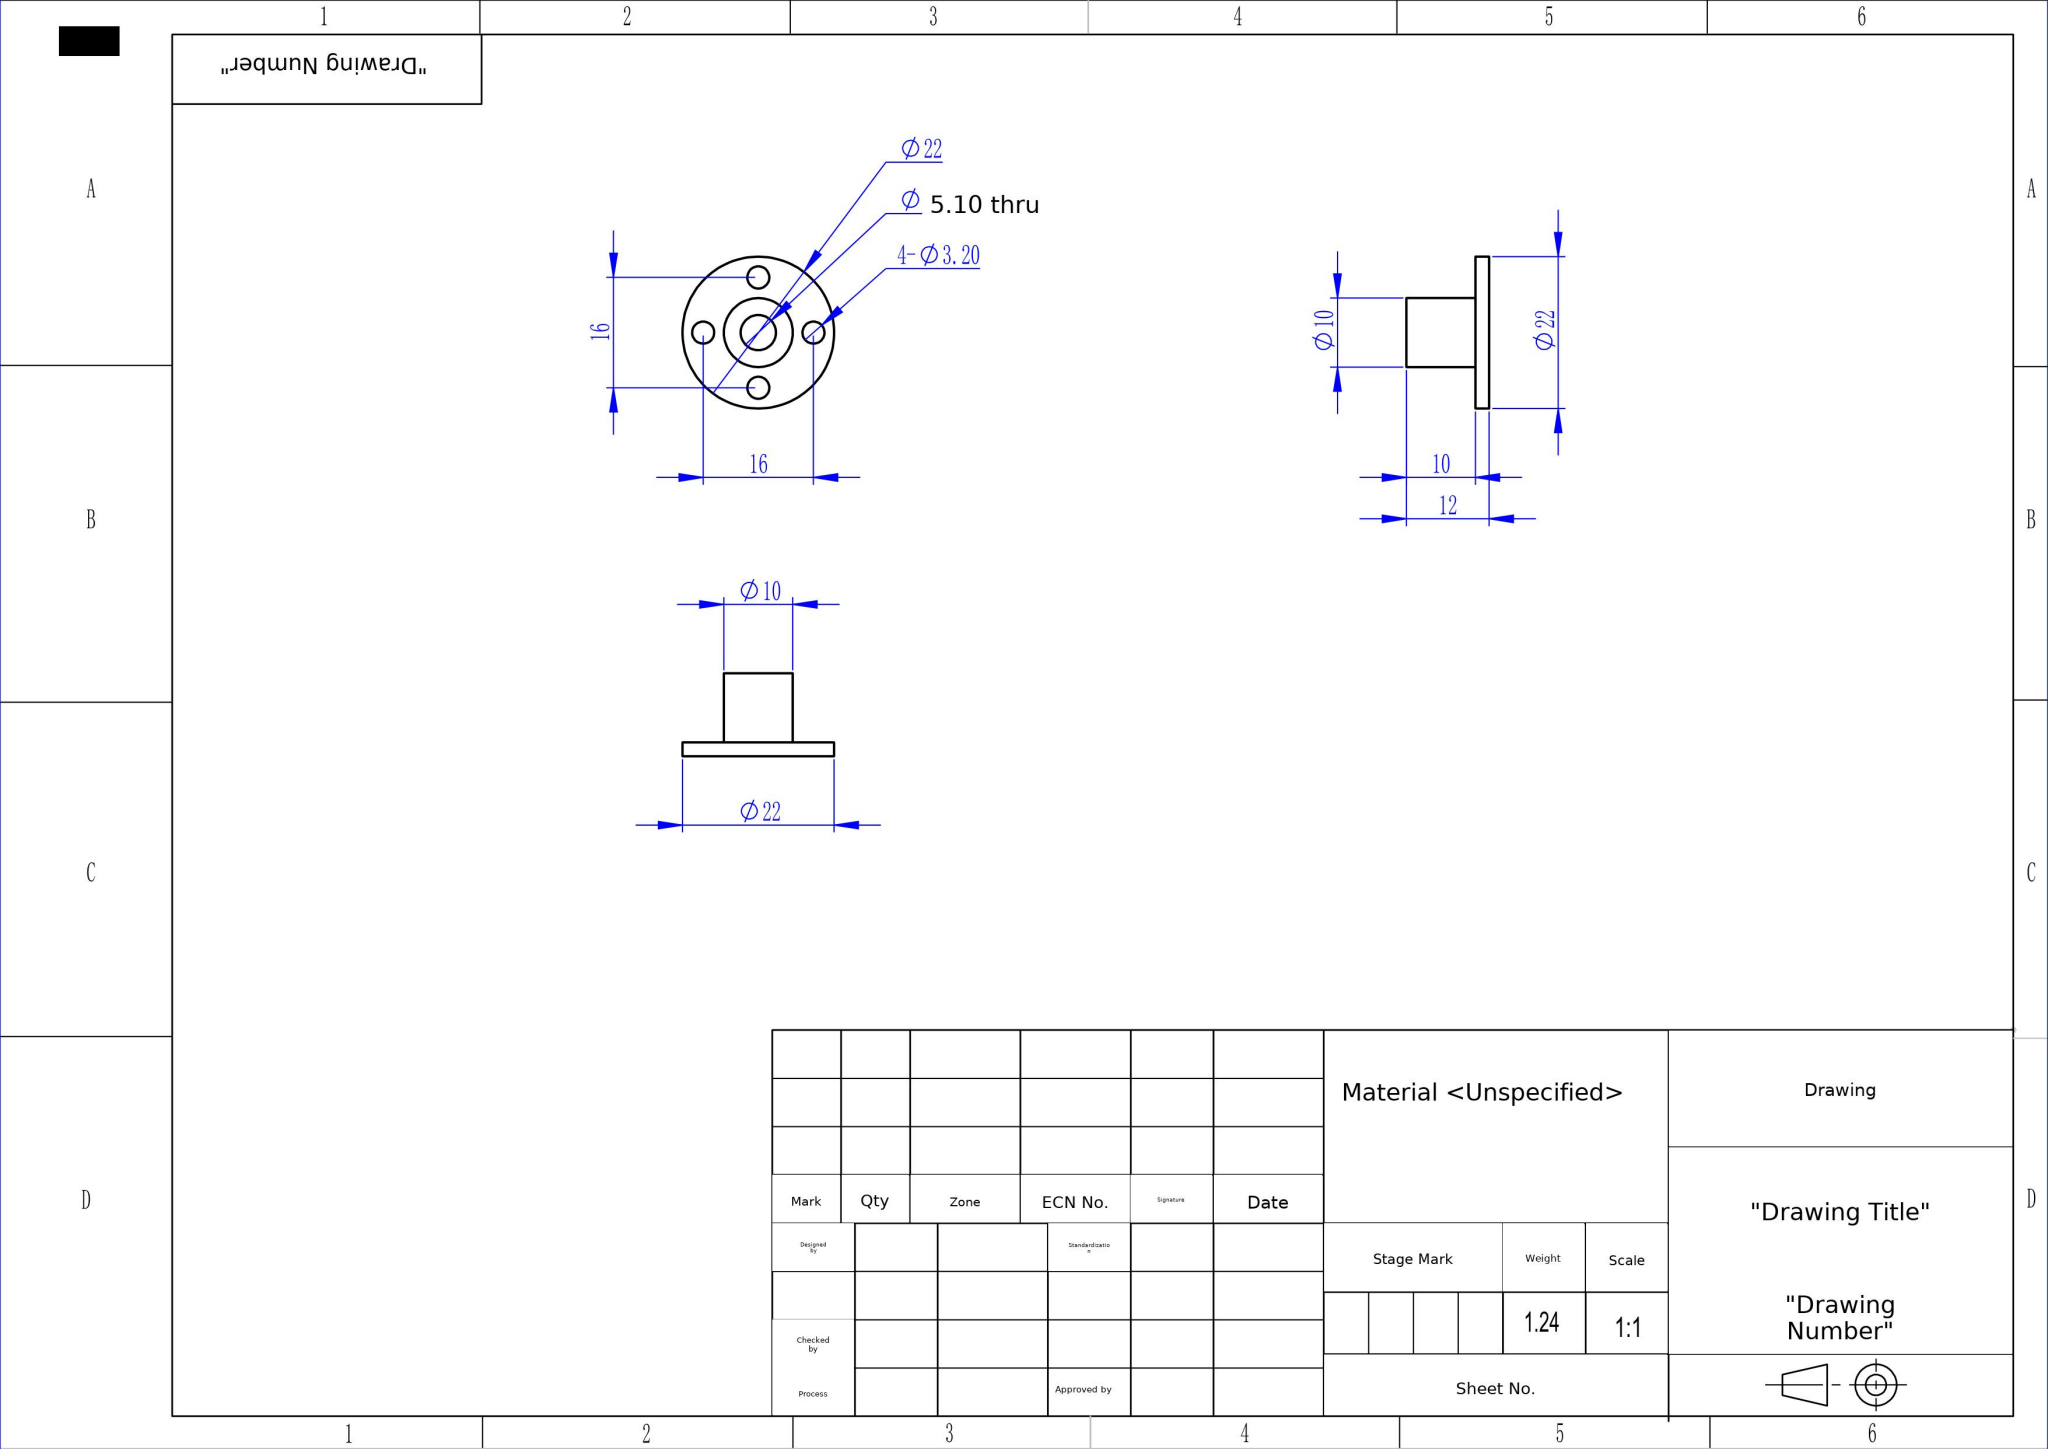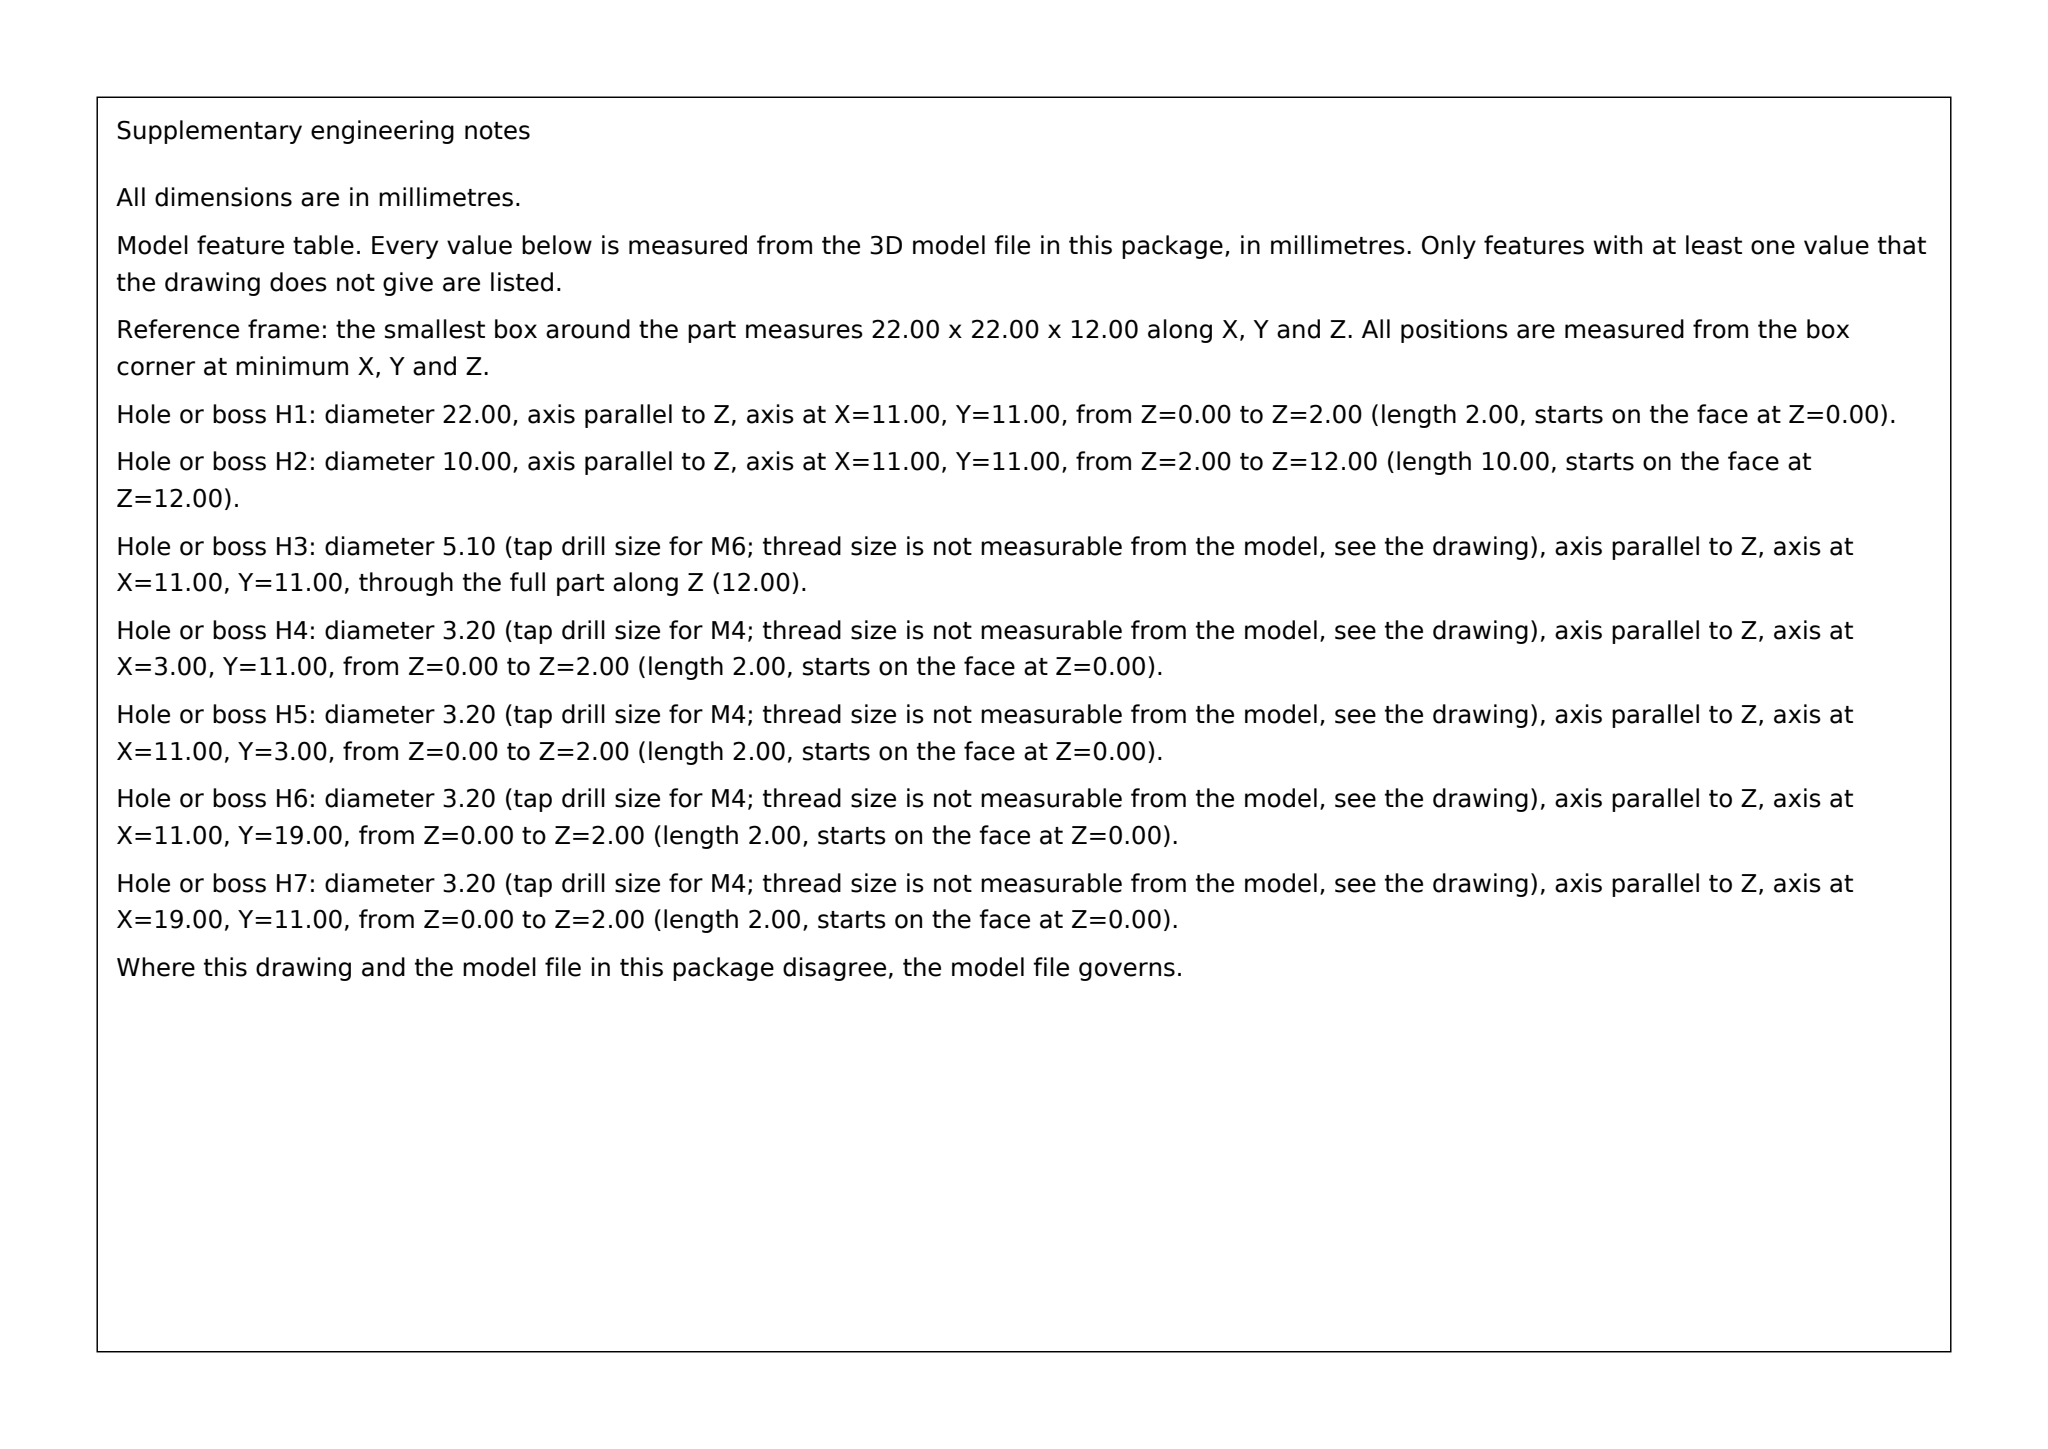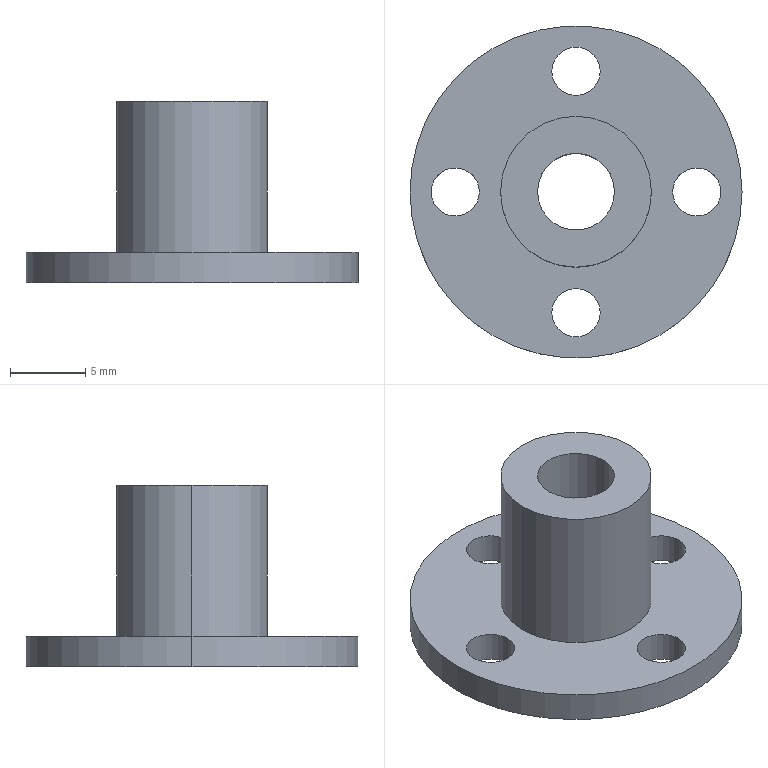Part | SolidWorks | mm | 1 solid | 17 faces | box 22 x 22 x 12 mm | volume 1236 mm3 | cylinder 14 | plane 3 | commonest cylinder face diameters 3.2 x8 5.1 x2 10 x2 22 x2
build123d program:
from build123d import *

# Parameters (mm, degrees)
SKETCH1_R           = 11
SKETCH1_R_2         = 1.6
BOSS_EXTRUDE1_DEPTH = 2
SKETCH2_R           = 5
BOSS_EXTRUDE2_DEPTH = 10
SKETCH3_R           = 2.55
CUT_EXTRUDE1_DEPTH  = 20.647


with BuildPart() as part:
    # Sketch1 → Boss-Extrude1 (new body)
    with BuildSketch(Plane.XY):
        Circle(SKETCH1_R)
        with Locations((-8, 0)):
            Circle(SKETCH1_R_2, mode=Mode.SUBTRACT)
        with Locations((8, 0)):
            Circle(SKETCH1_R_2, mode=Mode.SUBTRACT)
        with Locations((0, -8)):
            Circle(SKETCH1_R_2, mode=Mode.SUBTRACT)
        with Locations((0, 8)):
            Circle(SKETCH1_R_2, mode=Mode.SUBTRACT)
    extrude(amount=BOSS_EXTRUDE1_DEPTH)

    # Sketch2 → Boss-Extrude2 (add)
    with BuildSketch(Plane.XY.offset(2)):
        Circle(SKETCH2_R)
    extrude(amount=BOSS_EXTRUDE2_DEPTH)

    # Sketch3 → Cut-Extrude1 (cut, through all)
    with BuildSketch(Plane.XY.offset(12)):
        Circle(SKETCH3_R)
    extrude(amount=-CUT_EXTRUDE1_DEPTH, mode=Mode.SUBTRACT)


solid = part.part
STEP:
#1=CARTESIAN_POINT('',(-2.55,0.,0.));
#2=VERTEX_POINT('',#1);
#3=CARTESIAN_POINT('',(2.55,0.,0.));
#4=VERTEX_POINT('',#3);
#5=CARTESIAN_POINT('',(0.,0.,0.));
#6=DIRECTION('',(0.,0.,1.));
#7=DIRECTION('',(1.,0.,0.));
#8=AXIS2_PLACEMENT_3D('',#5,#6,#7);
#9=CIRCLE('',#8,2.55);
#10=EDGE_CURVE('',#2,#4,#9,.T.);
#11=ORIENTED_EDGE('',*,*,#10,.F.);
#12=CARTESIAN_POINT('',(-2.55,0.,12.));
#13=VERTEX_POINT('',#12);
#14=CARTESIAN_POINT('',(-2.55,0.,0.));
#15=DIRECTION('',(0.,0.,1.));
#16=VECTOR('',#15,1000.);
#17=LINE('',#14,#16);
#18=EDGE_CURVE('',#2,#13,#17,.T.);
#19=ORIENTED_EDGE('',*,*,#18,.T.);
#20=CARTESIAN_POINT('',(2.55,0.,12.));
#21=VERTEX_POINT('',#20);
#22=CARTESIAN_POINT('',(0.,0.,12.));
#23=DIRECTION('',(0.,0.,1.));
#24=DIRECTION('',(1.,0.,0.));
#25=AXIS2_PLACEMENT_3D('',#22,#23,#24);
#26=CIRCLE('',#25,2.55);
#27=EDGE_CURVE('',#13,#21,#26,.T.);
#28=ORIENTED_EDGE('',*,*,#27,.T.);
#29=CARTESIAN_POINT('',(2.55,0.,0.));
#30=DIRECTION('',(0.,0.,1.));
#31=VECTOR('',#30,1000.);
#32=LINE('',#29,#31);
#33=EDGE_CURVE('',#4,#21,#32,.T.);
#34=ORIENTED_EDGE('',*,*,#33,.F.);
#35=EDGE_LOOP('',(#11,#19,#28,#34));
#36=FACE_OUTER_BOUND('',#35,.T.);
#37=CARTESIAN_POINT('',(0.,0.,0.));
#38=DIRECTION('',(0.,0.,1.));
#39=DIRECTION('',(1.,0.,0.));
#40=AXIS2_PLACEMENT_3D('',#37,#38,#39);
#41=CYLINDRICAL_SURFACE('',#40,2.55);
#42=ADVANCED_FACE('',(#36),#41,.F.);
#43=CARTESIAN_POINT('',(5.,0.,12.));
#44=VERTEX_POINT('',#43);
#45=CARTESIAN_POINT('',(-5.,0.,12.));
#46=VERTEX_POINT('',#45);
#47=CARTESIAN_POINT('',(0.,0.,12.));
#48=DIRECTION('',(0.,0.,1.));
#49=DIRECTION('',(1.,0.,0.));
#50=AXIS2_PLACEMENT_3D('',#47,#48,#49);
#51=CIRCLE('',#50,5.);
#52=EDGE_CURVE('',#44,#46,#51,.T.);
#53=ORIENTED_EDGE('',*,*,#52,.F.);
#54=CARTESIAN_POINT('',(5.,0.,2.));
#55=VERTEX_POINT('',#54);
#56=CARTESIAN_POINT('',(5.,0.,12.));
#57=DIRECTION('',(0.,0.,-1.));
#58=VECTOR('',#57,1000.);
#59=LINE('',#56,#58);
#60=EDGE_CURVE('',#44,#55,#59,.T.);
#61=ORIENTED_EDGE('',*,*,#60,.T.);
#62=CARTESIAN_POINT('',(-5.,0.,2.));
#63=VERTEX_POINT('',#62);
#64=CARTESIAN_POINT('',(0.,0.,2.));
#65=DIRECTION('',(0.,0.,1.));
#66=DIRECTION('',(1.,0.,0.));
#67=AXIS2_PLACEMENT_3D('',#64,#65,#66);
#68=CIRCLE('',#67,5.);
#69=EDGE_CURVE('',#55,#63,#68,.T.);
#70=ORIENTED_EDGE('',*,*,#69,.T.);
#71=CARTESIAN_POINT('',(-5.,0.,12.));
#72=DIRECTION('',(0.,0.,-1.));
#73=VECTOR('',#72,1000.);
#74=LINE('',#71,#73);
#75=EDGE_CURVE('',#46,#63,#74,.T.);
#76=ORIENTED_EDGE('',*,*,#75,.F.);
#77=EDGE_LOOP('',(#53,#61,#70,#76));
#78=FACE_OUTER_BOUND('',#77,.T.);
#79=CARTESIAN_POINT('',(0.,0.,12.));
#80=DIRECTION('',(0.,0.,-1.));
#81=DIRECTION('',(-1.,0.,0.));
#82=AXIS2_PLACEMENT_3D('',#79,#80,#81);
#83=CYLINDRICAL_SURFACE('',#82,5.);
#84=ADVANCED_FACE('',(#78),#83,.T.);
#85=CARTESIAN_POINT('',(-1.6,8.,2.));
#86=VERTEX_POINT('',#85);
#87=CARTESIAN_POINT('',(1.6,8.,2.));
#88=VERTEX_POINT('',#87);
#89=CARTESIAN_POINT('',(0.,8.,2.));
#90=DIRECTION('',(0.,0.,1.));
#91=DIRECTION('',(1.,0.,0.));
#92=AXIS2_PLACEMENT_3D('',#89,#90,#91);
#93=CIRCLE('',#92,1.6);
#94=EDGE_CURVE('',#86,#88,#93,.T.);
#95=ORIENTED_EDGE('',*,*,#94,.T.);
#96=CARTESIAN_POINT('',(1.6,8.,0.));
#97=VERTEX_POINT('',#96);
#98=CARTESIAN_POINT('',(1.6,8.,2.));
#99=DIRECTION('',(0.,0.,-1.));
#100=VECTOR('',#99,1000.);
#101=LINE('',#98,#100);
#102=EDGE_CURVE('',#88,#97,#101,.T.);
#103=ORIENTED_EDGE('',*,*,#102,.T.);
#104=CARTESIAN_POINT('',(-1.6,8.,0.));
#105=VERTEX_POINT('',#104);
#106=CARTESIAN_POINT('',(0.,8.,0.));
#107=DIRECTION('',(0.,0.,1.));
#108=DIRECTION('',(1.,0.,0.));
#109=AXIS2_PLACEMENT_3D('',#106,#107,#108);
#110=CIRCLE('',#109,1.6);
#111=EDGE_CURVE('',#105,#97,#110,.T.);
#112=ORIENTED_EDGE('',*,*,#111,.F.);
#113=CARTESIAN_POINT('',(-1.6,8.,2.));
#114=DIRECTION('',(0.,0.,-1.));
#115=VECTOR('',#114,1000.);
#116=LINE('',#113,#115);
#117=EDGE_CURVE('',#86,#105,#116,.T.);
#118=ORIENTED_EDGE('',*,*,#117,.F.);
#119=EDGE_LOOP('',(#95,#103,#112,#118));
#120=FACE_OUTER_BOUND('',#119,.T.);
#121=CARTESIAN_POINT('',(0.,8.,2.));
#122=DIRECTION('',(0.,0.,-1.));
#123=DIRECTION('',(-1.,0.,0.));
#124=AXIS2_PLACEMENT_3D('',#121,#122,#123);
#125=CYLINDRICAL_SURFACE('',#124,1.6);
#126=ADVANCED_FACE('',(#120),#125,.F.);
#127=CARTESIAN_POINT('',(-1.6,-8.,2.));
#128=VERTEX_POINT('',#127);
#129=CARTESIAN_POINT('',(1.6,-8.,2.));
#130=VERTEX_POINT('',#129);
#131=CARTESIAN_POINT('',(0.,-8.,2.));
#132=DIRECTION('',(0.,0.,1.));
#133=DIRECTION('',(1.,0.,0.));
#134=AXIS2_PLACEMENT_3D('',#131,#132,#133);
#135=CIRCLE('',#134,1.6);
#136=EDGE_CURVE('',#128,#130,#135,.T.);
#137=ORIENTED_EDGE('',*,*,#136,.T.);
#138=CARTESIAN_POINT('',(1.6,-8.,0.));
#139=VERTEX_POINT('',#138);
#140=CARTESIAN_POINT('',(1.6,-8.,2.));
#141=DIRECTION('',(0.,0.,-1.));
#142=VECTOR('',#141,1000.);
#143=LINE('',#140,#142);
#144=EDGE_CURVE('',#130,#139,#143,.T.);
#145=ORIENTED_EDGE('',*,*,#144,.T.);
#146=CARTESIAN_POINT('',(-1.6,-8.,0.));
#147=VERTEX_POINT('',#146);
#148=CARTESIAN_POINT('',(0.,-8.,0.));
#149=DIRECTION('',(0.,0.,1.));
#150=DIRECTION('',(1.,0.,0.));
#151=AXIS2_PLACEMENT_3D('',#148,#149,#150);
#152=CIRCLE('',#151,1.6);
#153=EDGE_CURVE('',#147,#139,#152,.T.);
#154=ORIENTED_EDGE('',*,*,#153,.F.);
#155=CARTESIAN_POINT('',(-1.6,-8.,2.));
#156=DIRECTION('',(0.,0.,-1.));
#157=VECTOR('',#156,1000.);
#158=LINE('',#155,#157);
#159=EDGE_CURVE('',#128,#147,#158,.T.);
#160=ORIENTED_EDGE('',*,*,#159,.F.);
#161=EDGE_LOOP('',(#137,#145,#154,#160));
#162=FACE_OUTER_BOUND('',#161,.T.);
#163=CARTESIAN_POINT('',(0.,-8.,2.));
#164=DIRECTION('',(0.,0.,-1.));
#165=DIRECTION('',(-1.,0.,0.));
#166=AXIS2_PLACEMENT_3D('',#163,#164,#165);
#167=CYLINDRICAL_SURFACE('',#166,1.6);
#168=ADVANCED_FACE('',(#162),#167,.F.);
#169=CARTESIAN_POINT('',(6.4,0.,2.));
#170=VERTEX_POINT('',#169);
#171=CARTESIAN_POINT('',(9.6,0.,2.));
#172=VERTEX_POINT('',#171);
#173=CARTESIAN_POINT('',(8.,0.,2.));
#174=DIRECTION('',(0.,0.,1.));
#175=DIRECTION('',(1.,0.,0.));
#176=AXIS2_PLACEMENT_3D('',#173,#174,#175);
#177=CIRCLE('',#176,1.6);
#178=EDGE_CURVE('',#170,#172,#177,.T.);
#179=ORIENTED_EDGE('',*,*,#178,.T.);
#180=CARTESIAN_POINT('',(9.6,0.,0.));
#181=VERTEX_POINT('',#180);
#182=CARTESIAN_POINT('',(9.6,0.,2.));
#183=DIRECTION('',(0.,0.,-1.));
#184=VECTOR('',#183,1000.);
#185=LINE('',#182,#184);
#186=EDGE_CURVE('',#172,#181,#185,.T.);
#187=ORIENTED_EDGE('',*,*,#186,.T.);
#188=CARTESIAN_POINT('',(6.4,0.,0.));
#189=VERTEX_POINT('',#188);
#190=CARTESIAN_POINT('',(8.,0.,0.));
#191=DIRECTION('',(0.,0.,1.));
#192=DIRECTION('',(1.,0.,0.));
#193=AXIS2_PLACEMENT_3D('',#190,#191,#192);
#194=CIRCLE('',#193,1.6);
#195=EDGE_CURVE('',#189,#181,#194,.T.);
#196=ORIENTED_EDGE('',*,*,#195,.F.);
#197=CARTESIAN_POINT('',(6.4,0.,2.));
#198=DIRECTION('',(0.,0.,-1.));
#199=VECTOR('',#198,1000.);
#200=LINE('',#197,#199);
#201=EDGE_CURVE('',#170,#189,#200,.T.);
#202=ORIENTED_EDGE('',*,*,#201,.F.);
#203=EDGE_LOOP('',(#179,#187,#196,#202));
#204=FACE_OUTER_BOUND('',#203,.T.);
#205=CARTESIAN_POINT('',(8.,0.,2.));
#206=DIRECTION('',(0.,0.,-1.));
#207=DIRECTION('',(-1.,0.,0.));
#208=AXIS2_PLACEMENT_3D('',#205,#206,#207);
#209=CYLINDRICAL_SURFACE('',#208,1.6);
#210=ADVANCED_FACE('',(#204),#209,.F.);
#211=CARTESIAN_POINT('',(-9.6,0.,2.));
#212=VERTEX_POINT('',#211);
#213=CARTESIAN_POINT('',(-6.4,0.,2.));
#214=VERTEX_POINT('',#213);
#215=CARTESIAN_POINT('',(-8.,0.,2.));
#216=DIRECTION('',(0.,0.,1.));
#217=DIRECTION('',(1.,0.,0.));
#218=AXIS2_PLACEMENT_3D('',#215,#216,#217);
#219=CIRCLE('',#218,1.6);
#220=EDGE_CURVE('',#212,#214,#219,.T.);
#221=ORIENTED_EDGE('',*,*,#220,.T.);
#222=CARTESIAN_POINT('',(-6.4,0.,0.));
#223=VERTEX_POINT('',#222);
#224=CARTESIAN_POINT('',(-6.4,0.,2.));
#225=DIRECTION('',(0.,0.,-1.));
#226=VECTOR('',#225,1000.);
#227=LINE('',#224,#226);
#228=EDGE_CURVE('',#214,#223,#227,.T.);
#229=ORIENTED_EDGE('',*,*,#228,.T.);
#230=CARTESIAN_POINT('',(-9.6,0.,0.));
#231=VERTEX_POINT('',#230);
#232=CARTESIAN_POINT('',(-8.,0.,0.));
#233=DIRECTION('',(0.,0.,1.));
#234=DIRECTION('',(1.,0.,0.));
#235=AXIS2_PLACEMENT_3D('',#232,#233,#234);
#236=CIRCLE('',#235,1.6);
#237=EDGE_CURVE('',#231,#223,#236,.T.);
#238=ORIENTED_EDGE('',*,*,#237,.F.);
#239=CARTESIAN_POINT('',(-9.6,0.,2.));
#240=DIRECTION('',(0.,0.,-1.));
#241=VECTOR('',#240,1000.);
#242=LINE('',#239,#241);
#243=EDGE_CURVE('',#212,#231,#242,.T.);
#244=ORIENTED_EDGE('',*,*,#243,.F.);
#245=EDGE_LOOP('',(#221,#229,#238,#244));
#246=FACE_OUTER_BOUND('',#245,.T.);
#247=CARTESIAN_POINT('',(-8.,0.,2.));
#248=DIRECTION('',(0.,0.,-1.));
#249=DIRECTION('',(-1.,0.,0.));
#250=AXIS2_PLACEMENT_3D('',#247,#248,#249);
#251=CYLINDRICAL_SURFACE('',#250,1.6);
#252=ADVANCED_FACE('',(#246),#251,.F.);
#253=CARTESIAN_POINT('',(11.,0.,2.));
#254=VERTEX_POINT('',#253);
#255=CARTESIAN_POINT('',(-11.,0.,2.));
#256=VERTEX_POINT('',#255);
#257=CARTESIAN_POINT('',(0.,0.,2.));
#258=DIRECTION('',(0.,0.,1.));
#259=DIRECTION('',(1.,0.,0.));
#260=AXIS2_PLACEMENT_3D('',#257,#258,#259);
#261=CIRCLE('',#260,11.);
#262=EDGE_CURVE('',#254,#256,#261,.T.);
#263=ORIENTED_EDGE('',*,*,#262,.F.);
#264=CARTESIAN_POINT('',(11.,0.,0.));
#265=VERTEX_POINT('',#264);
#266=CARTESIAN_POINT('',(11.,0.,2.));
#267=DIRECTION('',(0.,0.,-1.));
#268=VECTOR('',#267,1000.);
#269=LINE('',#266,#268);
#270=EDGE_CURVE('',#254,#265,#269,.T.);
#271=ORIENTED_EDGE('',*,*,#270,.T.);
#272=CARTESIAN_POINT('',(-11.,0.,0.));
#273=VERTEX_POINT('',#272);
#274=CARTESIAN_POINT('',(0.,0.,0.));
#275=DIRECTION('',(0.,0.,1.));
#276=DIRECTION('',(1.,0.,0.));
#277=AXIS2_PLACEMENT_3D('',#274,#275,#276);
#278=CIRCLE('',#277,11.);
#279=EDGE_CURVE('',#265,#273,#278,.T.);
#280=ORIENTED_EDGE('',*,*,#279,.T.);
#281=CARTESIAN_POINT('',(-11.,0.,2.));
#282=DIRECTION('',(0.,0.,-1.));
#283=VECTOR('',#282,1000.);
#284=LINE('',#281,#283);
#285=EDGE_CURVE('',#256,#273,#284,.T.);
#286=ORIENTED_EDGE('',*,*,#285,.F.);
#287=EDGE_LOOP('',(#263,#271,#280,#286));
#288=FACE_OUTER_BOUND('',#287,.T.);
#289=CARTESIAN_POINT('',(0.,0.,2.));
#290=DIRECTION('',(0.,0.,-1.));
#291=DIRECTION('',(-1.,0.,0.));
#292=AXIS2_PLACEMENT_3D('',#289,#290,#291);
#293=CYLINDRICAL_SURFACE('',#292,11.);
#294=ADVANCED_FACE('',(#288),#293,.T.);
#295=CARTESIAN_POINT('',(0.,0.,2.));
#296=DIRECTION('',(0.,0.,1.));
#297=DIRECTION('',(1.,0.,0.));
#298=AXIS2_PLACEMENT_3D('',#295,#296,#297);
#299=CIRCLE('',#298,5.);
#300=EDGE_CURVE('',#63,#55,#299,.T.);
#301=ORIENTED_EDGE('',*,*,#300,.F.);
#302=ORIENTED_EDGE('',*,*,#69,.F.);
#303=EDGE_LOOP('',(#301,#302));
#304=FACE_BOUND('',#303,.T.);
#305=ORIENTED_EDGE('',*,*,#136,.F.);
#306=CARTESIAN_POINT('',(0.,-8.,2.));
#307=DIRECTION('',(0.,0.,1.));
#308=DIRECTION('',(1.,0.,0.));
#309=AXIS2_PLACEMENT_3D('',#306,#307,#308);
#310=CIRCLE('',#309,1.6);
#311=EDGE_CURVE('',#130,#128,#310,.T.);
#312=ORIENTED_EDGE('',*,*,#311,.F.);
#313=EDGE_LOOP('',(#305,#312));
#314=FACE_BOUND('',#313,.T.);
#315=ORIENTED_EDGE('',*,*,#220,.F.);
#316=CARTESIAN_POINT('',(-8.,0.,2.));
#317=DIRECTION('',(0.,0.,1.));
#318=DIRECTION('',(1.,0.,0.));
#319=AXIS2_PLACEMENT_3D('',#316,#317,#318);
#320=CIRCLE('',#319,1.6);
#321=EDGE_CURVE('',#214,#212,#320,.T.);
#322=ORIENTED_EDGE('',*,*,#321,.F.);
#323=EDGE_LOOP('',(#315,#322));
#324=FACE_BOUND('',#323,.T.);
#325=CARTESIAN_POINT('',(0.,0.,2.));
#326=DIRECTION('',(0.,0.,1.));
#327=DIRECTION('',(1.,0.,0.));
#328=AXIS2_PLACEMENT_3D('',#325,#326,#327);
#329=CIRCLE('',#328,11.);
#330=EDGE_CURVE('',#256,#254,#329,.T.);
#331=ORIENTED_EDGE('',*,*,#330,.T.);
#332=ORIENTED_EDGE('',*,*,#262,.T.);
#333=EDGE_LOOP('',(#331,#332));
#334=FACE_OUTER_BOUND('',#333,.T.);
#335=ORIENTED_EDGE('',*,*,#178,.F.);
#336=CARTESIAN_POINT('',(8.,0.,2.));
#337=DIRECTION('',(0.,0.,1.));
#338=DIRECTION('',(1.,0.,0.));
#339=AXIS2_PLACEMENT_3D('',#336,#337,#338);
#340=CIRCLE('',#339,1.6);
#341=EDGE_CURVE('',#172,#170,#340,.T.);
#342=ORIENTED_EDGE('',*,*,#341,.F.);
#343=EDGE_LOOP('',(#335,#342));
#344=FACE_BOUND('',#343,.T.);
#345=ORIENTED_EDGE('',*,*,#94,.F.);
#346=CARTESIAN_POINT('',(0.,8.,2.));
#347=DIRECTION('',(0.,0.,1.));
#348=DIRECTION('',(1.,0.,0.));
#349=AXIS2_PLACEMENT_3D('',#346,#347,#348);
#350=CIRCLE('',#349,1.6);
#351=EDGE_CURVE('',#88,#86,#350,.T.);
#352=ORIENTED_EDGE('',*,*,#351,.F.);
#353=EDGE_LOOP('',(#345,#352));
#354=FACE_BOUND('',#353,.T.);
#355=CARTESIAN_POINT('',(0.,0.,2.));
#356=DIRECTION('',(0.,0.,1.));
#357=DIRECTION('',(1.,0.,0.));
#358=AXIS2_PLACEMENT_3D('',#355,#356,#357);
#359=PLANE('',#358);
#360=ADVANCED_FACE('',(#304,#314,#324,#334,#344,#354),#359,.T.);
#361=CARTESIAN_POINT('',(0.,0.,0.));
#362=DIRECTION('',(0.,0.,1.));
#363=DIRECTION('',(1.,0.,0.));
#364=AXIS2_PLACEMENT_3D('',#361,#362,#363);
#365=CIRCLE('',#364,2.55);
#366=EDGE_CURVE('',#4,#2,#365,.T.);
#367=ORIENTED_EDGE('',*,*,#366,.T.);
#368=ORIENTED_EDGE('',*,*,#10,.T.);
#369=EDGE_LOOP('',(#367,#368));
#370=FACE_BOUND('',#369,.T.);
#371=CARTESIAN_POINT('',(0.,0.,0.));
#372=DIRECTION('',(0.,0.,1.));
#373=DIRECTION('',(1.,0.,0.));
#374=AXIS2_PLACEMENT_3D('',#371,#372,#373);
#375=CIRCLE('',#374,11.);
#376=EDGE_CURVE('',#273,#265,#375,.T.);
#377=ORIENTED_EDGE('',*,*,#376,.F.);
#378=ORIENTED_EDGE('',*,*,#279,.F.);
#379=EDGE_LOOP('',(#377,#378));
#380=FACE_OUTER_BOUND('',#379,.T.);
#381=ORIENTED_EDGE('',*,*,#237,.T.);
#382=CARTESIAN_POINT('',(-8.,0.,0.));
#383=DIRECTION('',(0.,0.,1.));
#384=DIRECTION('',(1.,0.,0.));
#385=AXIS2_PLACEMENT_3D('',#382,#383,#384);
#386=CIRCLE('',#385,1.6);
#387=EDGE_CURVE('',#223,#231,#386,.T.);
#388=ORIENTED_EDGE('',*,*,#387,.T.);
#389=EDGE_LOOP('',(#381,#388));
#390=FACE_BOUND('',#389,.T.);
#391=ORIENTED_EDGE('',*,*,#195,.T.);
#392=CARTESIAN_POINT('',(8.,0.,0.));
#393=DIRECTION('',(0.,0.,1.));
#394=DIRECTION('',(1.,0.,0.));
#395=AXIS2_PLACEMENT_3D('',#392,#393,#394);
#396=CIRCLE('',#395,1.6);
#397=EDGE_CURVE('',#181,#189,#396,.T.);
#398=ORIENTED_EDGE('',*,*,#397,.T.);
#399=EDGE_LOOP('',(#391,#398));
#400=FACE_BOUND('',#399,.T.);
#401=ORIENTED_EDGE('',*,*,#153,.T.);
#402=CARTESIAN_POINT('',(0.,-8.,0.));
#403=DIRECTION('',(0.,0.,1.));
#404=DIRECTION('',(1.,0.,0.));
#405=AXIS2_PLACEMENT_3D('',#402,#403,#404);
#406=CIRCLE('',#405,1.6);
#407=EDGE_CURVE('',#139,#147,#406,.T.);
#408=ORIENTED_EDGE('',*,*,#407,.T.);
#409=EDGE_LOOP('',(#401,#408));
#410=FACE_BOUND('',#409,.T.);
#411=ORIENTED_EDGE('',*,*,#111,.T.);
#412=CARTESIAN_POINT('',(0.,8.,0.));
#413=DIRECTION('',(0.,0.,1.));
#414=DIRECTION('',(1.,0.,0.));
#415=AXIS2_PLACEMENT_3D('',#412,#413,#414);
#416=CIRCLE('',#415,1.6);
#417=EDGE_CURVE('',#97,#105,#416,.T.);
#418=ORIENTED_EDGE('',*,*,#417,.T.);
#419=EDGE_LOOP('',(#411,#418));
#420=FACE_BOUND('',#419,.T.);
#421=CARTESIAN_POINT('',(0.,0.,0.));
#422=DIRECTION('',(0.,0.,1.));
#423=DIRECTION('',(1.,0.,0.));
#424=AXIS2_PLACEMENT_3D('',#421,#422,#423);
#425=PLANE('',#424);
#426=ADVANCED_FACE('',(#370,#380,#390,#400,#410,#420),#425,.F.);
#427=ORIENTED_EDGE('',*,*,#270,.F.);
#428=ORIENTED_EDGE('',*,*,#330,.F.);
#429=ORIENTED_EDGE('',*,*,#285,.T.);
#430=ORIENTED_EDGE('',*,*,#376,.T.);
#431=EDGE_LOOP('',(#427,#428,#429,#430));
#432=FACE_OUTER_BOUND('',#431,.T.);
#433=CARTESIAN_POINT('',(0.,0.,2.));
#434=DIRECTION('',(0.,0.,-1.));
#435=DIRECTION('',(-1.,0.,0.));
#436=AXIS2_PLACEMENT_3D('',#433,#434,#435);
#437=CYLINDRICAL_SURFACE('',#436,11.);
#438=ADVANCED_FACE('',(#432),#437,.T.);
#439=ORIENTED_EDGE('',*,*,#228,.F.);
#440=ORIENTED_EDGE('',*,*,#321,.T.);
#441=ORIENTED_EDGE('',*,*,#243,.T.);
#442=ORIENTED_EDGE('',*,*,#387,.F.);
#443=EDGE_LOOP('',(#439,#440,#441,#442));
#444=FACE_OUTER_BOUND('',#443,.T.);
#445=CARTESIAN_POINT('',(-8.,0.,2.));
#446=DIRECTION('',(0.,0.,-1.));
#447=DIRECTION('',(-1.,0.,0.));
#448=AXIS2_PLACEMENT_3D('',#445,#446,#447);
#449=CYLINDRICAL_SURFACE('',#448,1.6);
#450=ADVANCED_FACE('',(#444),#449,.F.);
#451=ORIENTED_EDGE('',*,*,#186,.F.);
#452=ORIENTED_EDGE('',*,*,#341,.T.);
#453=ORIENTED_EDGE('',*,*,#201,.T.);
#454=ORIENTED_EDGE('',*,*,#397,.F.);
#455=EDGE_LOOP('',(#451,#452,#453,#454));
#456=FACE_OUTER_BOUND('',#455,.T.);
#457=CARTESIAN_POINT('',(8.,0.,2.));
#458=DIRECTION('',(0.,0.,-1.));
#459=DIRECTION('',(-1.,0.,0.));
#460=AXIS2_PLACEMENT_3D('',#457,#458,#459);
#461=CYLINDRICAL_SURFACE('',#460,1.6);
#462=ADVANCED_FACE('',(#456),#461,.F.);
#463=ORIENTED_EDGE('',*,*,#144,.F.);
#464=ORIENTED_EDGE('',*,*,#311,.T.);
#465=ORIENTED_EDGE('',*,*,#159,.T.);
#466=ORIENTED_EDGE('',*,*,#407,.F.);
#467=EDGE_LOOP('',(#463,#464,#465,#466));
#468=FACE_OUTER_BOUND('',#467,.T.);
#469=CARTESIAN_POINT('',(0.,-8.,2.));
#470=DIRECTION('',(0.,0.,-1.));
#471=DIRECTION('',(-1.,0.,0.));
#472=AXIS2_PLACEMENT_3D('',#469,#470,#471);
#473=CYLINDRICAL_SURFACE('',#472,1.6);
#474=ADVANCED_FACE('',(#468),#473,.F.);
#475=ORIENTED_EDGE('',*,*,#102,.F.);
#476=ORIENTED_EDGE('',*,*,#351,.T.);
#477=ORIENTED_EDGE('',*,*,#117,.T.);
#478=ORIENTED_EDGE('',*,*,#417,.F.);
#479=EDGE_LOOP('',(#475,#476,#477,#478));
#480=FACE_OUTER_BOUND('',#479,.T.);
#481=CARTESIAN_POINT('',(0.,8.,2.));
#482=DIRECTION('',(0.,0.,-1.));
#483=DIRECTION('',(-1.,0.,0.));
#484=AXIS2_PLACEMENT_3D('',#481,#482,#483);
#485=CYLINDRICAL_SURFACE('',#484,1.6);
#486=ADVANCED_FACE('',(#480),#485,.F.);
#487=ORIENTED_EDGE('',*,*,#60,.F.);
#488=CARTESIAN_POINT('',(0.,0.,12.));
#489=DIRECTION('',(0.,0.,1.));
#490=DIRECTION('',(1.,0.,0.));
#491=AXIS2_PLACEMENT_3D('',#488,#489,#490);
#492=CIRCLE('',#491,5.);
#493=EDGE_CURVE('',#46,#44,#492,.T.);
#494=ORIENTED_EDGE('',*,*,#493,.F.);
#495=ORIENTED_EDGE('',*,*,#75,.T.);
#496=ORIENTED_EDGE('',*,*,#300,.T.);
#497=EDGE_LOOP('',(#487,#494,#495,#496));
#498=FACE_OUTER_BOUND('',#497,.T.);
#499=CARTESIAN_POINT('',(0.,0.,12.));
#500=DIRECTION('',(0.,0.,-1.));
#501=DIRECTION('',(-1.,0.,0.));
#502=AXIS2_PLACEMENT_3D('',#499,#500,#501);
#503=CYLINDRICAL_SURFACE('',#502,5.);
#504=ADVANCED_FACE('',(#498),#503,.T.);
#505=CARTESIAN_POINT('',(0.,0.,12.));
#506=DIRECTION('',(0.,0.,1.));
#507=DIRECTION('',(1.,0.,0.));
#508=AXIS2_PLACEMENT_3D('',#505,#506,#507);
#509=CIRCLE('',#508,2.55);
#510=EDGE_CURVE('',#21,#13,#509,.T.);
#511=ORIENTED_EDGE('',*,*,#510,.F.);
#512=ORIENTED_EDGE('',*,*,#27,.F.);
#513=EDGE_LOOP('',(#511,#512));
#514=FACE_BOUND('',#513,.T.);
#515=ORIENTED_EDGE('',*,*,#493,.T.);
#516=ORIENTED_EDGE('',*,*,#52,.T.);
#517=EDGE_LOOP('',(#515,#516));
#518=FACE_OUTER_BOUND('',#517,.T.);
#519=CARTESIAN_POINT('',(0.,0.,12.));
#520=DIRECTION('',(0.,0.,1.));
#521=DIRECTION('',(1.,0.,0.));
#522=AXIS2_PLACEMENT_3D('',#519,#520,#521);
#523=PLANE('',#522);
#524=ADVANCED_FACE('',(#514,#518),#523,.T.);
#525=ORIENTED_EDGE('',*,*,#18,.F.);
#526=ORIENTED_EDGE('',*,*,#366,.F.);
#527=ORIENTED_EDGE('',*,*,#33,.T.);
#528=ORIENTED_EDGE('',*,*,#510,.T.);
#529=EDGE_LOOP('',(#525,#526,#527,#528));
#530=FACE_OUTER_BOUND('',#529,.T.);
#531=CARTESIAN_POINT('',(0.,0.,0.));
#532=DIRECTION('',(0.,0.,1.));
#533=DIRECTION('',(1.,0.,0.));
#534=AXIS2_PLACEMENT_3D('',#531,#532,#533);
#535=CYLINDRICAL_SURFACE('',#534,2.55);
#536=ADVANCED_FACE('',(#530),#535,.F.);
#537=CLOSED_SHELL('',(#42,#84,#126,#168,#210,#252,#294,#360,#426,#438,#450,#462,#474,#486,#504,#524,#536));
#538=MANIFOLD_SOLID_BREP('',#537);
#539=CARTESIAN_POINT('',(0.,0.,0.));
#540=DIRECTION('',(0.,0.,1.));
#541=DIRECTION('',(1.,0.,0.));
#542=AXIS2_PLACEMENT_3D('',#539,#540,#541);
#543=(LENGTH_UNIT()NAMED_UNIT(*)SI_UNIT(.MILLI.,.METRE.));
#544=UNCERTAINTY_MEASURE_WITH_UNIT(LENGTH_MEASURE(0.00001),#543,'','');
#545=(NAMED_UNIT(*)PLANE_ANGLE_UNIT()SI_UNIT($,.RADIAN.));
#546=(NAMED_UNIT(*)SI_UNIT($,.STERADIAN.)SOLID_ANGLE_UNIT());
#547=(GEOMETRIC_REPRESENTATION_CONTEXT(3)GLOBAL_UNCERTAINTY_ASSIGNED_CONTEXT((#544))GLOBAL_UNIT_ASSIGNED_CONTEXT((#543,#545,#546))REPRESENTATION_CONTEXT('',''));
#548=ADVANCED_BREP_SHAPE_REPRESENTATION('',(#538,#542),#547);